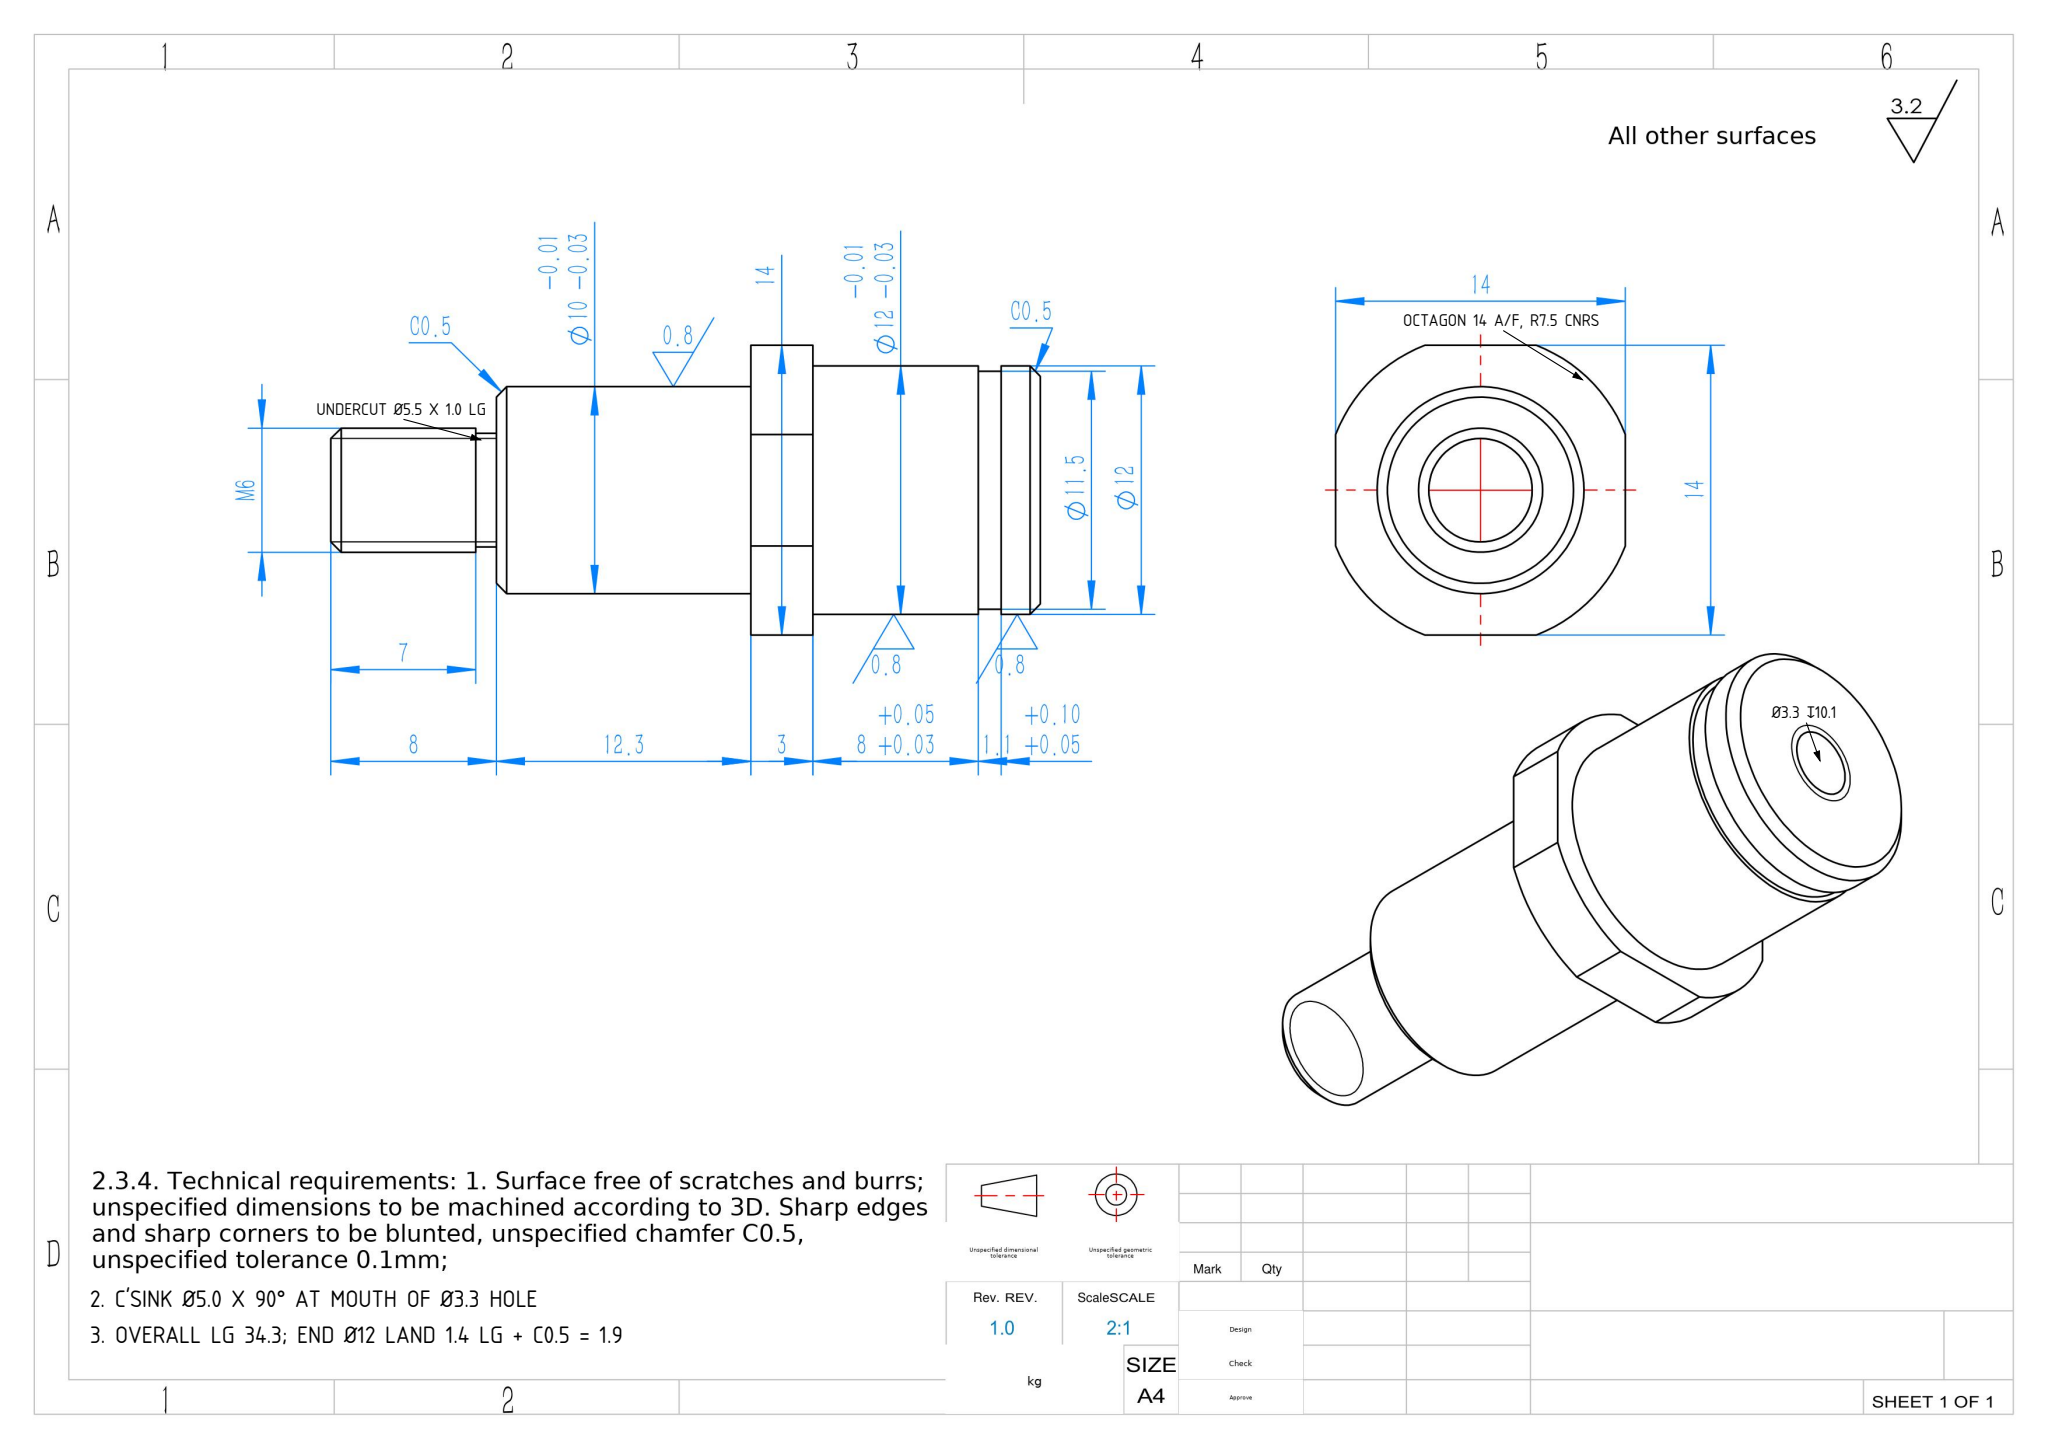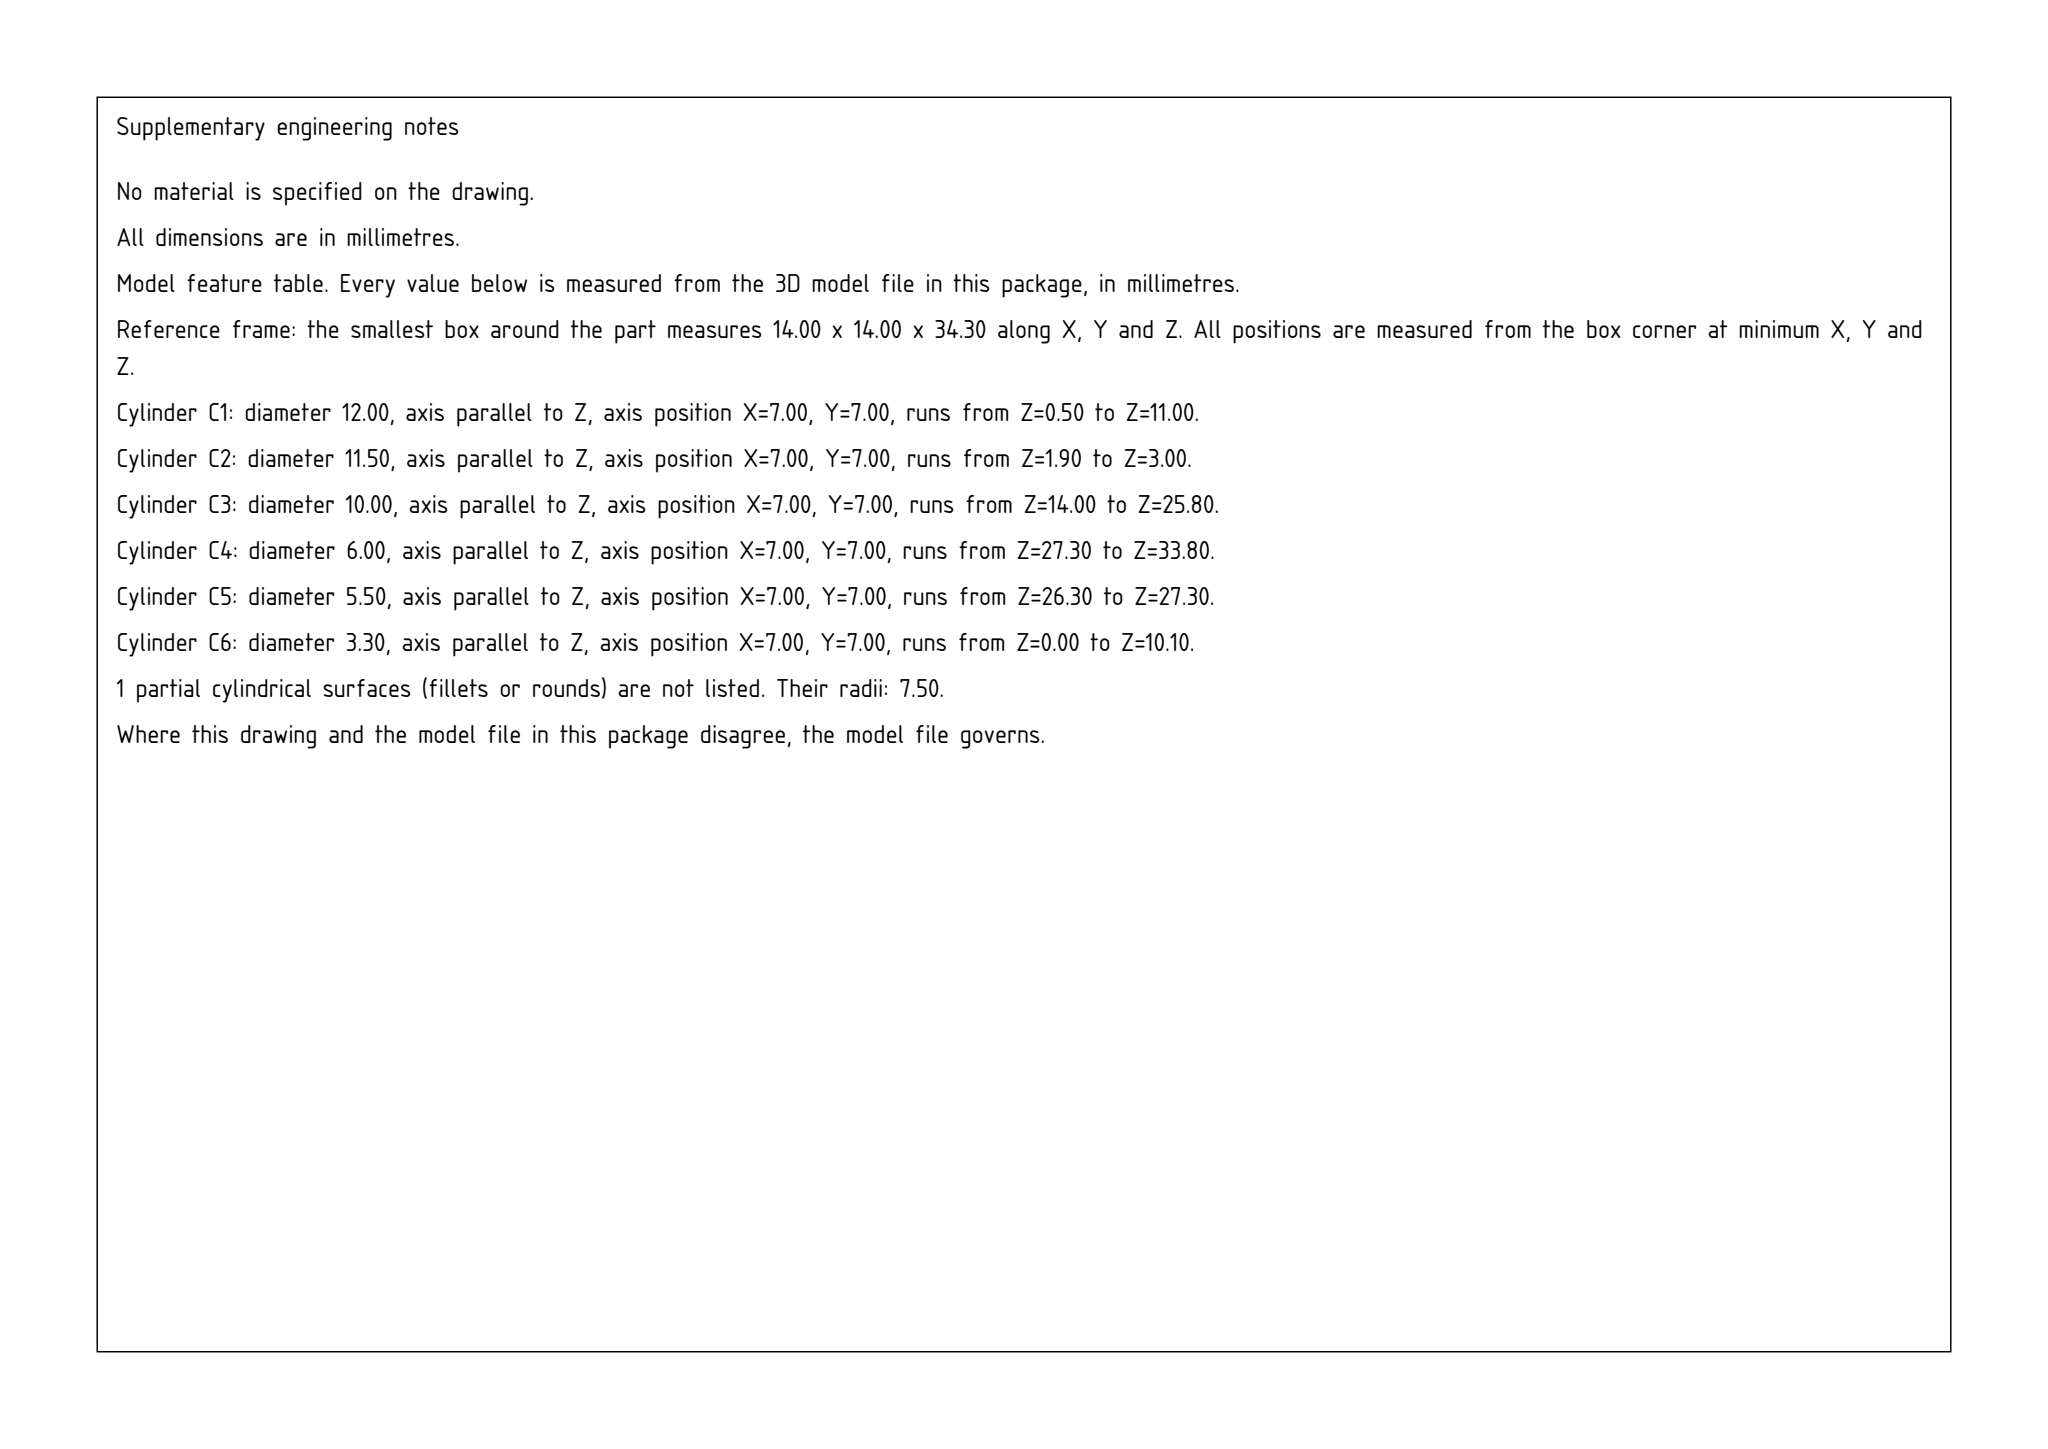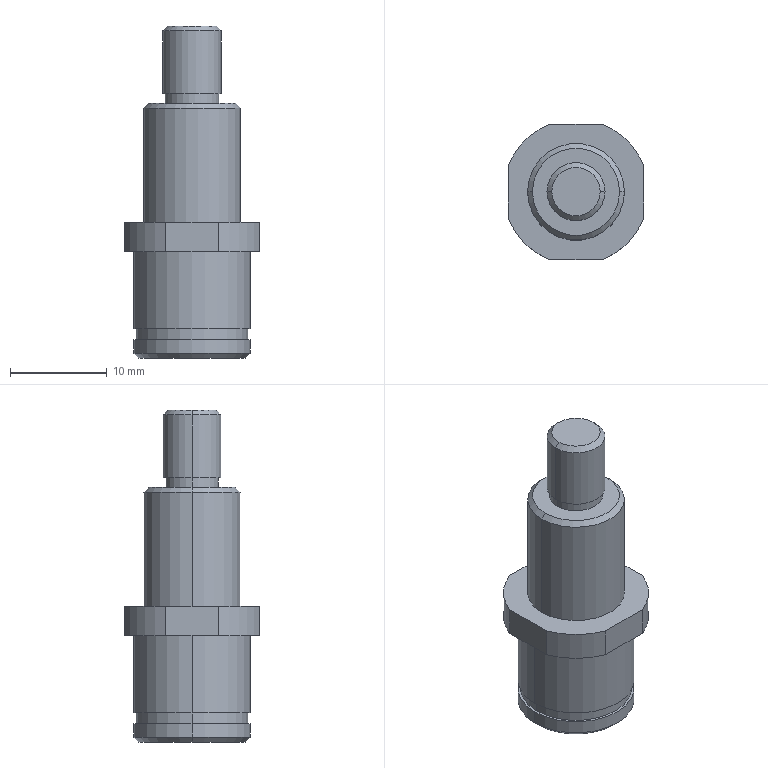Part | SolidWorks | mm | 1 solid | 38 faces | box 14 x 14 x 34.3 mm | volume 2830 mm3 | cylinder 18 | plane 12 | cone 8 | commonest cylinder face diameters 12 x4 15 x4 6 x2 5.5 x2 3.3 x2 11.5 x2 10 x2
Drawing notes:
CENTRAL HOLE Ø3.3 DP 10.1 FROM Ø12 END FACE | from the solid: cyl dia 3.3 axis z at (7,7), length 10.1, starts at z=0 end face (Ø12 land)
C'SINK Ø5.0 X 90° AT MOUTH OF Ø3.3 HOLE | from the solid: cone included angle 90.0, ref dia 5.0, at z=0 mouth of Ø3.3 bore
OVERALL LG 34.3; END Ø12 LAND 1.4 LG + C0.5 = 1.9 | from the solid: bbox z 34.3; cyl Ø12 length 1.4 from z=0; z-plane at 1.9 after C0.5 (cone 90°, ref dia 11.0)
THD UNDERCUT Ø5.5 X 1.0 LG BEHIND M6 | from the solid: cyl dia 5.5 axis z, length 1.0, between z=26.3 and 27.3, ahead of Ø6 M6 thread
OCTAGON HEAD 3 LG: 14 A/F, CORNERS R7.5 (Ø15) | from the solid: planes x=0/14, y=0/14 (14 across flats) + 4 cyl dia 15.0 axis z, length 3.0, z=11.0 to 14.0
build123d program:
from build123d import *

# Parameters (mm, degrees)
SKETCH1_R             = 7.5
BOSS_EXTRUDE1_DEPTH   = 3
SKETCH2_R             = 5
BOSS_EXTRUDE2_DEPTH   = 12.3
SKETCH3_R             = 3
BOSS_EXTRUDE3_DEPTH   = 8
CHAMFER1_SIZE         = 0.5
SKETCH4_R             = 6
BOSS_EXTRUDE4_DEPTH   = 11
SKETCH5_W             = 1.041
SKETCH5_H             = 1.1
CHAMFER2_SIZE         = 0.5
M4_TAPPED_HOLE1_D     = 3.3
M4_TAPPED_HOLE1_DEPTH = 10.1
M4_TAPPED_HOLE1_TIP   = 0.9914
SKETCH8_OUTSIDE_W     = 25.066
SKETCH8_OUTSIDE_H     = 25.066
SKETCH8_OUTSIDE_W_2   = 14
SKETCH8_OUTSIDE_H_2   = 14
CUT_EXTRUDE1_DEPTH    = 10
CHAMFER3_SIZE         = 0.5
SKETCH9_OUTSIDE_W     = 23.92
SKETCH9_OUTSIDE_H     = 23.92
SKETCH9_OUTSIDE_R     = 2.75
CUT_EXTRUDE2_DEPTH    = 1


with BuildPart() as part:
    # Sketch1 → Boss-Extrude1 (new body)
    with BuildSketch(Plane.XY):
        Circle(SKETCH1_R)
    extrude(amount=BOSS_EXTRUDE1_DEPTH)

    # Sketch2 → Boss-Extrude2 (add)
    with BuildSketch(Plane.XY.offset(3)):
        Circle(SKETCH2_R)
    extrude(amount=BOSS_EXTRUDE2_DEPTH)

    # Sketch3 → Boss-Extrude3 (add)
    with BuildSketch(Plane.XY.offset(15.3)):
        Circle(SKETCH3_R)
    extrude(amount=BOSS_EXTRUDE3_DEPTH)

    # Chamfer1
    chamfer1_edges = [part.edges().sort_by_distance(p)[0] for p in [
        (-3, 0, 23.3),
    ]]
    chamfer(chamfer1_edges, length=CHAMFER1_SIZE)

    # Sketch4 → Boss-Extrude4 (add)
    with BuildSketch(Plane(origin=(0, 0, 0), x_dir=(-1, 0, 0), z_dir=(0, 0, -1))):
        Circle(SKETCH4_R)
    extrude(amount=BOSS_EXTRUDE4_DEPTH)

    # Sketch5 → Cut-Revolve1 (revolve, cut)
    with BuildSketch(Plane(origin=(0, 0, 0), x_dir=(1, 0, 0), z_dir=(0, 1, 0))):
        with Locations((6.27, 8.55)):
            Rectangle(SKETCH5_W, SKETCH5_H)
    revolve(axis=Axis((0, 0, 0), (0, 0, -1)), mode=Mode.SUBTRACT)

    # Chamfer2
    chamfer2_edges = [part.edges().sort_by_distance(p)[0] for p in [
        (6, 0, -11),
    ]]
    chamfer(chamfer2_edges, length=CHAMFER2_SIZE)

    # M4 Tapped Hole1
    with Locations(Plane(origin=(0, 0, -11), x_dir=(-1, 0, 0), z_dir=(0, 0, -1))):
        with Locations((0, 0)):
            Hole(M4_TAPPED_HOLE1_D / 2, depth=M4_TAPPED_HOLE1_DEPTH)
            with Locations((0, 0, -(M4_TAPPED_HOLE1_DEPTH + M4_TAPPED_HOLE1_TIP / 2))):  # 118° drill point
                Cone(0, M4_TAPPED_HOLE1_D / 2, M4_TAPPED_HOLE1_TIP, mode=Mode.SUBTRACT)

    # Sketch8 outside → Cut-Extrude1 (cut)
    with BuildSketch(Plane(origin=(0, 0, 0), x_dir=(-1, 0, 0), z_dir=(0, 0, -1))):
        Rectangle(SKETCH8_OUTSIDE_W, SKETCH8_OUTSIDE_H)
        Rectangle(SKETCH8_OUTSIDE_W_2, SKETCH8_OUTSIDE_H_2, mode=Mode.SUBTRACT)
    extrude(amount=-CUT_EXTRUDE1_DEPTH, mode=Mode.SUBTRACT)

    # Chamfer3
    chamfer3_edges = [part.edges().sort_by_distance(p)[0] for p in [
        (-5, 0, 15.3),
    ]]
    chamfer(chamfer3_edges, length=CHAMFER3_SIZE)

    # Sketch9 outside → Cut-Extrude2 (cut)
    with BuildSketch(Plane.XY.offset(15.3)):
        Rectangle(SKETCH9_OUTSIDE_W, SKETCH9_OUTSIDE_H)
        Circle(SKETCH9_OUTSIDE_R, mode=Mode.SUBTRACT)
    extrude(amount=CUT_EXTRUDE2_DEPTH, mode=Mode.SUBTRACT)


solid = part.part